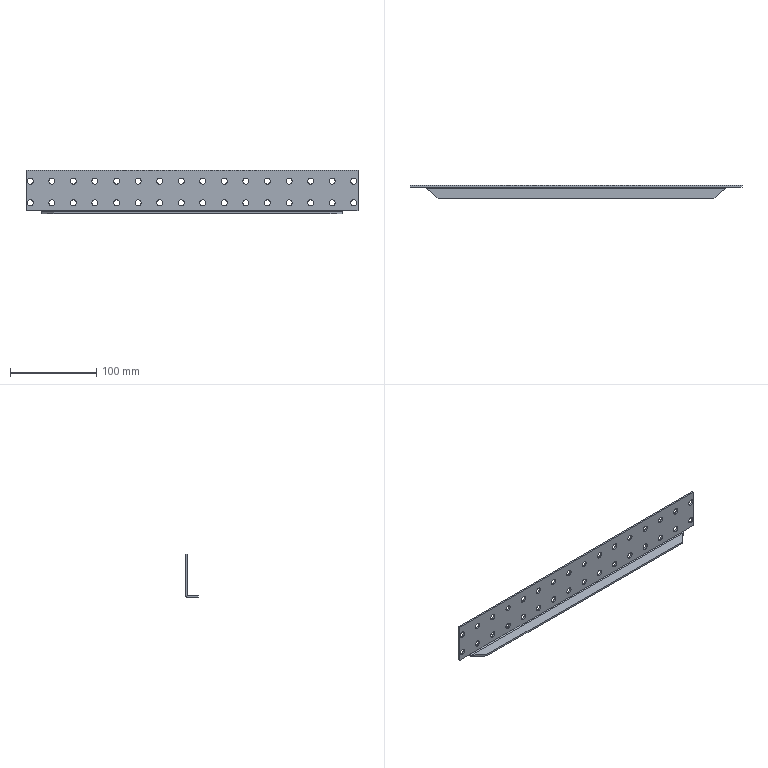Component | SolidWorks | Beam(No.26)-2 | 1 solid | 80 faces | volume 43931 mm3 | cylinder 66 | plane 12 | spline 2 | commonest cylinder face diameters 7 x64 6 x1 2 x1